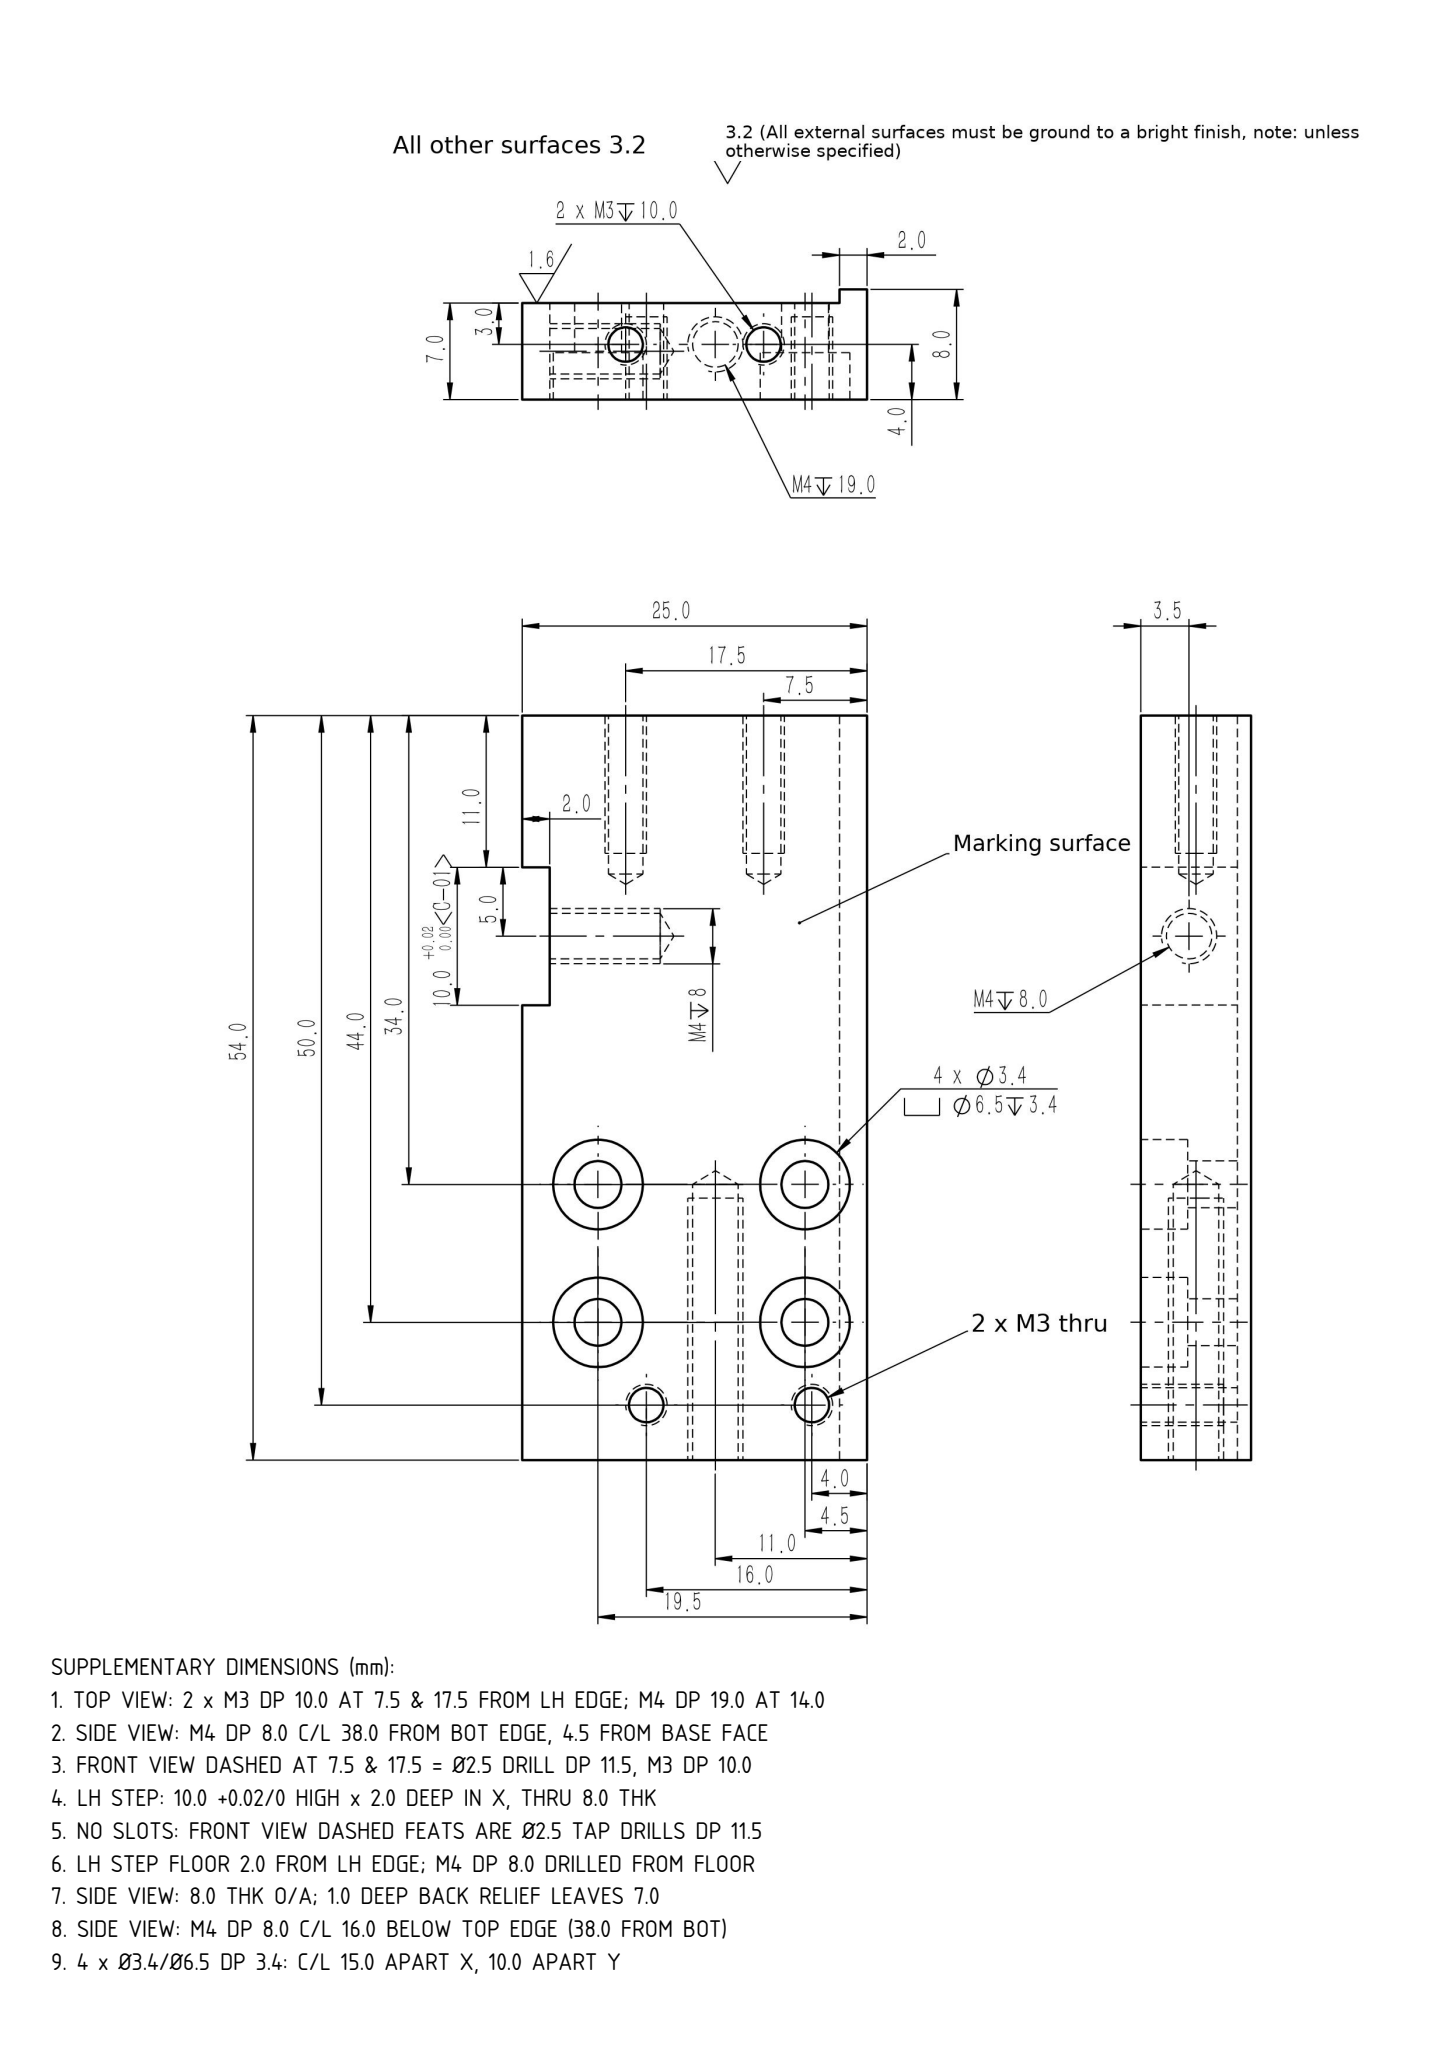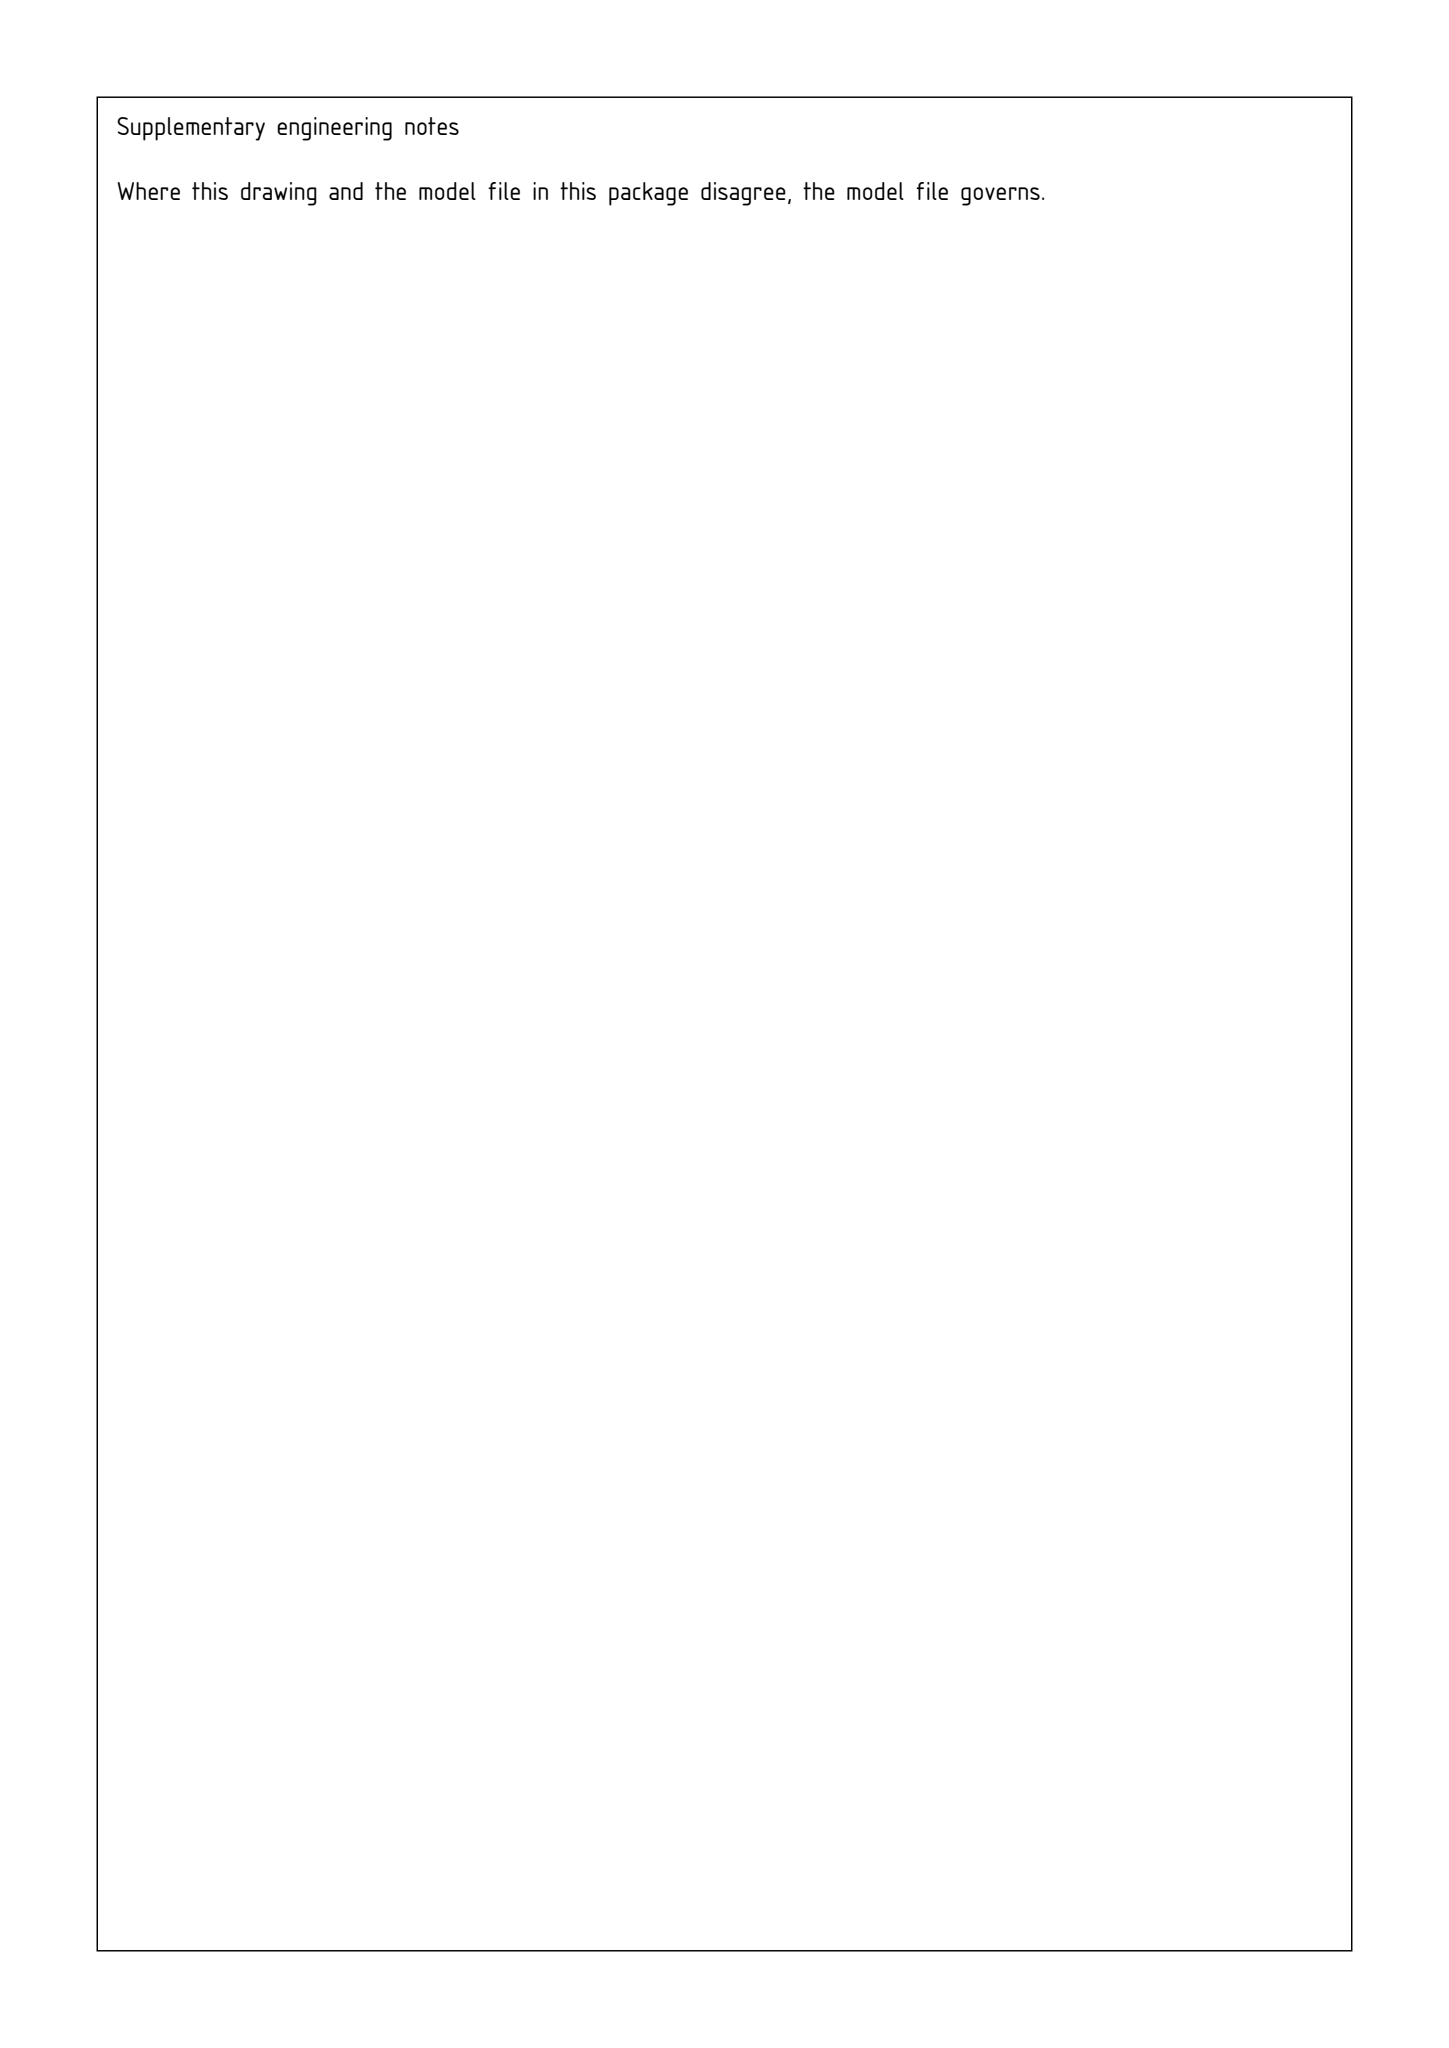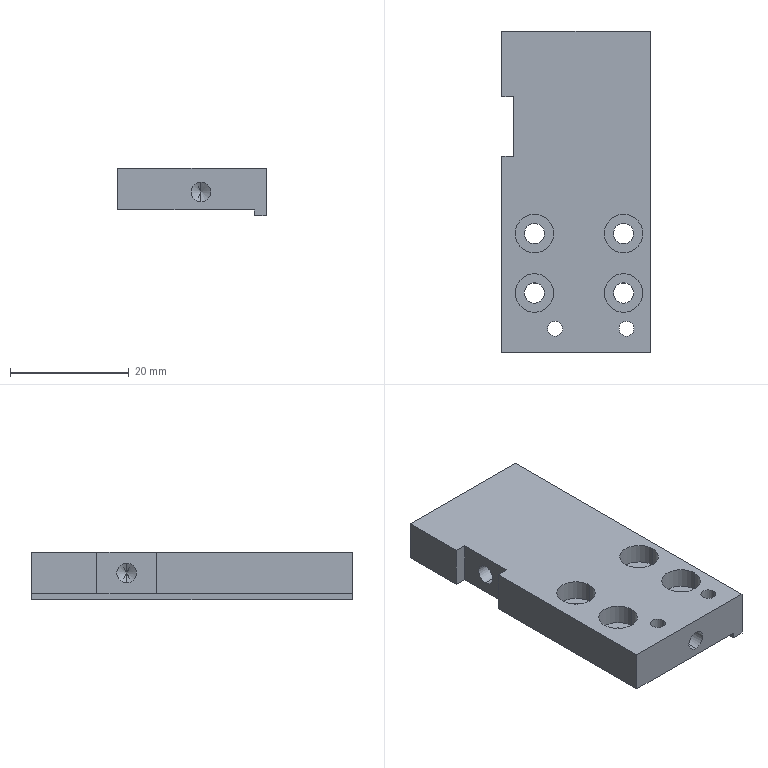Part | SolidWorks | mm | 1 solid | 52 faces | box 25 x 54 x 8 mm | volume 8407 mm3 | cylinder 28 | plane 16 | cone 8 | commonest cylinder face diameters 2.5 x8 6.5 x8 3.4 x8 3.3 x4
build123d program:
from build123d import *

# Parameters (mm, degrees)
SKETCH1_W                                       = 25
SKETCH1_H                                       = 54
BOSS_EXTRUDE1_DEPTH                             = 8
SKETCH2_W                                       = 23
SKETCH2_H                                       = 54
CUT_EXTRUDE1_DEPTH                              = 1
M3_HEX_SOCKET_HEAD_CAP_SCREW_CBORE1_D           = 3.4
M3_HEX_SOCKET_HEAD_CAP_SCREW_CBORE1_CBORE_D     = 6.5
M3_HEX_SOCKET_HEAD_CAP_SCREW_CBORE1_CBORE_DEPTH = 3.4
LPATTERN1_COUNT                                 = 2
LPATTERN1_PITCH                                 = 10
LPATTERN1_COUNT_DIR2                            = 2
LPATTERN1_PITCH_DIR2                            = 15
M3_TAPPED_HOLE1_D                               = 2.5
M3_TAPPED_HOLE1_DEPTH                           = 7.5
M3_TAPPED_HOLE1_TIP                             = 0.7511
M4_TAPPED_HOLE2_D                               = 3.3
M4_TAPPED_HOLE2_DEPTH                           = 20
M4_TAPPED_HOLE2_TIP                             = 0.9914
M3_TAPPED_HOLE2_D                               = 2.5
M3_TAPPED_HOLE2_DEPTH                           = 11.5
M3_TAPPED_HOLE2_TIP                             = 0.7511
SKETCH14_W                                      = 7
SKETCH14_H                                      = 10
CUT_EXTRUDE2_DEPTH                              = 2
M4_TAPPED_HOLE3_D                               = 3.3
M4_TAPPED_HOLE3_DEPTH                           = 8
M4_TAPPED_HOLE3_TIP                             = 0.9914


with BuildPart() as part:
    # Sketch1 → Boss-Extrude1 (new body)
    with BuildSketch(Plane.XY):
        with Locations((12.5, 27)):
            Rectangle(SKETCH1_W, SKETCH1_H)
    extrude(amount=BOSS_EXTRUDE1_DEPTH)

    # Sketch2 → Cut-Extrude1 (cut)
    with BuildSketch(Plane(origin=(0, 0, 0), x_dir=(-1, 0, 0), z_dir=(0, 0, -1))):
        with Locations((-11.5, 27)):
            Rectangle(SKETCH2_W, SKETCH2_H)
    extrude(amount=-CUT_EXTRUDE1_DEPTH, mode=Mode.SUBTRACT)

    # M3 Hex Socket Head Cap Screw CBORE1 (through all)
    with Locations(Plane.XY.offset(8)):
        with Locations((5.5, 10)):
            m3_hex_socket_head_cap_screw_cbore1 = CounterBoreHole(M3_HEX_SOCKET_HEAD_CAP_SCREW_CBORE1_D / 2, M3_HEX_SOCKET_HEAD_CAP_SCREW_CBORE1_CBORE_D / 2, M3_HEX_SOCKET_HEAD_CAP_SCREW_CBORE1_CBORE_DEPTH)

    # LPattern1: M3 Hex Socket Head Cap Screw CBORE1 2 × 2
    with Locations(*[(j * LPATTERN1_PITCH_DIR2, i * LPATTERN1_PITCH, 0) for i in range(LPATTERN1_COUNT) for j in range(LPATTERN1_COUNT_DIR2) if (i, j) != (0, 0)]):
        add(m3_hex_socket_head_cap_screw_cbore1, mode=Mode.SUBTRACT)

    # M3 Tapped Hole1
    with Locations(Plane.XY.offset(8)):
        with Locations((21, 4), (9, 4)):
            Hole(M3_TAPPED_HOLE1_D / 2, depth=M3_TAPPED_HOLE1_DEPTH)
            with Locations((0, 0, -(M3_TAPPED_HOLE1_DEPTH + M3_TAPPED_HOLE1_TIP / 2))):  # 118° drill point
                Cone(0, M3_TAPPED_HOLE1_D / 2, M3_TAPPED_HOLE1_TIP, mode=Mode.SUBTRACT)

    # M4 Tapped Hole2
    with Locations(Plane(origin=(0, 0, 0), x_dir=(-1, 0, 0), z_dir=(0, -1, 0))):
        with Locations((-14, -4)):
            Hole(M4_TAPPED_HOLE2_D / 2, depth=M4_TAPPED_HOLE2_DEPTH)
            with Locations((0, 0, -(M4_TAPPED_HOLE2_DEPTH + M4_TAPPED_HOLE2_TIP / 2))):  # 118° drill point
                Cone(0, M4_TAPPED_HOLE2_D / 2, M4_TAPPED_HOLE2_TIP, mode=Mode.SUBTRACT)

    # M3 Tapped Hole2
    with Locations(Plane(origin=(0, 54, 0), x_dir=(1, 0, 0), z_dir=(0, 1, 0))):
        with Locations((7.5, -4), (17.5, -4)):
            Hole(M3_TAPPED_HOLE2_D / 2, depth=M3_TAPPED_HOLE2_DEPTH)
            with Locations((0, 0, -(M3_TAPPED_HOLE2_DEPTH + M3_TAPPED_HOLE2_TIP / 2))):  # 118° drill point
                Cone(0, M3_TAPPED_HOLE2_D / 2, M3_TAPPED_HOLE2_TIP, mode=Mode.SUBTRACT)

    # Sketch14 → Cut-Extrude2 (cut)
    with BuildSketch(Plane.ZY):
        with Locations((4.5, 38)):
            Rectangle(SKETCH14_W, SKETCH14_H)
    extrude(amount=-CUT_EXTRUDE2_DEPTH, mode=Mode.SUBTRACT)

    # M4 Tapped Hole3
    with Locations(Plane.ZY.offset(-2)):
        with Locations((4.5, 38)):
            Hole(M4_TAPPED_HOLE3_D / 2, depth=M4_TAPPED_HOLE3_DEPTH)
            with Locations((0, 0, -(M4_TAPPED_HOLE3_DEPTH + M4_TAPPED_HOLE3_TIP / 2))):  # 118° drill point
                Cone(0, M4_TAPPED_HOLE3_D / 2, M4_TAPPED_HOLE3_TIP, mode=Mode.SUBTRACT)


solid = part.part